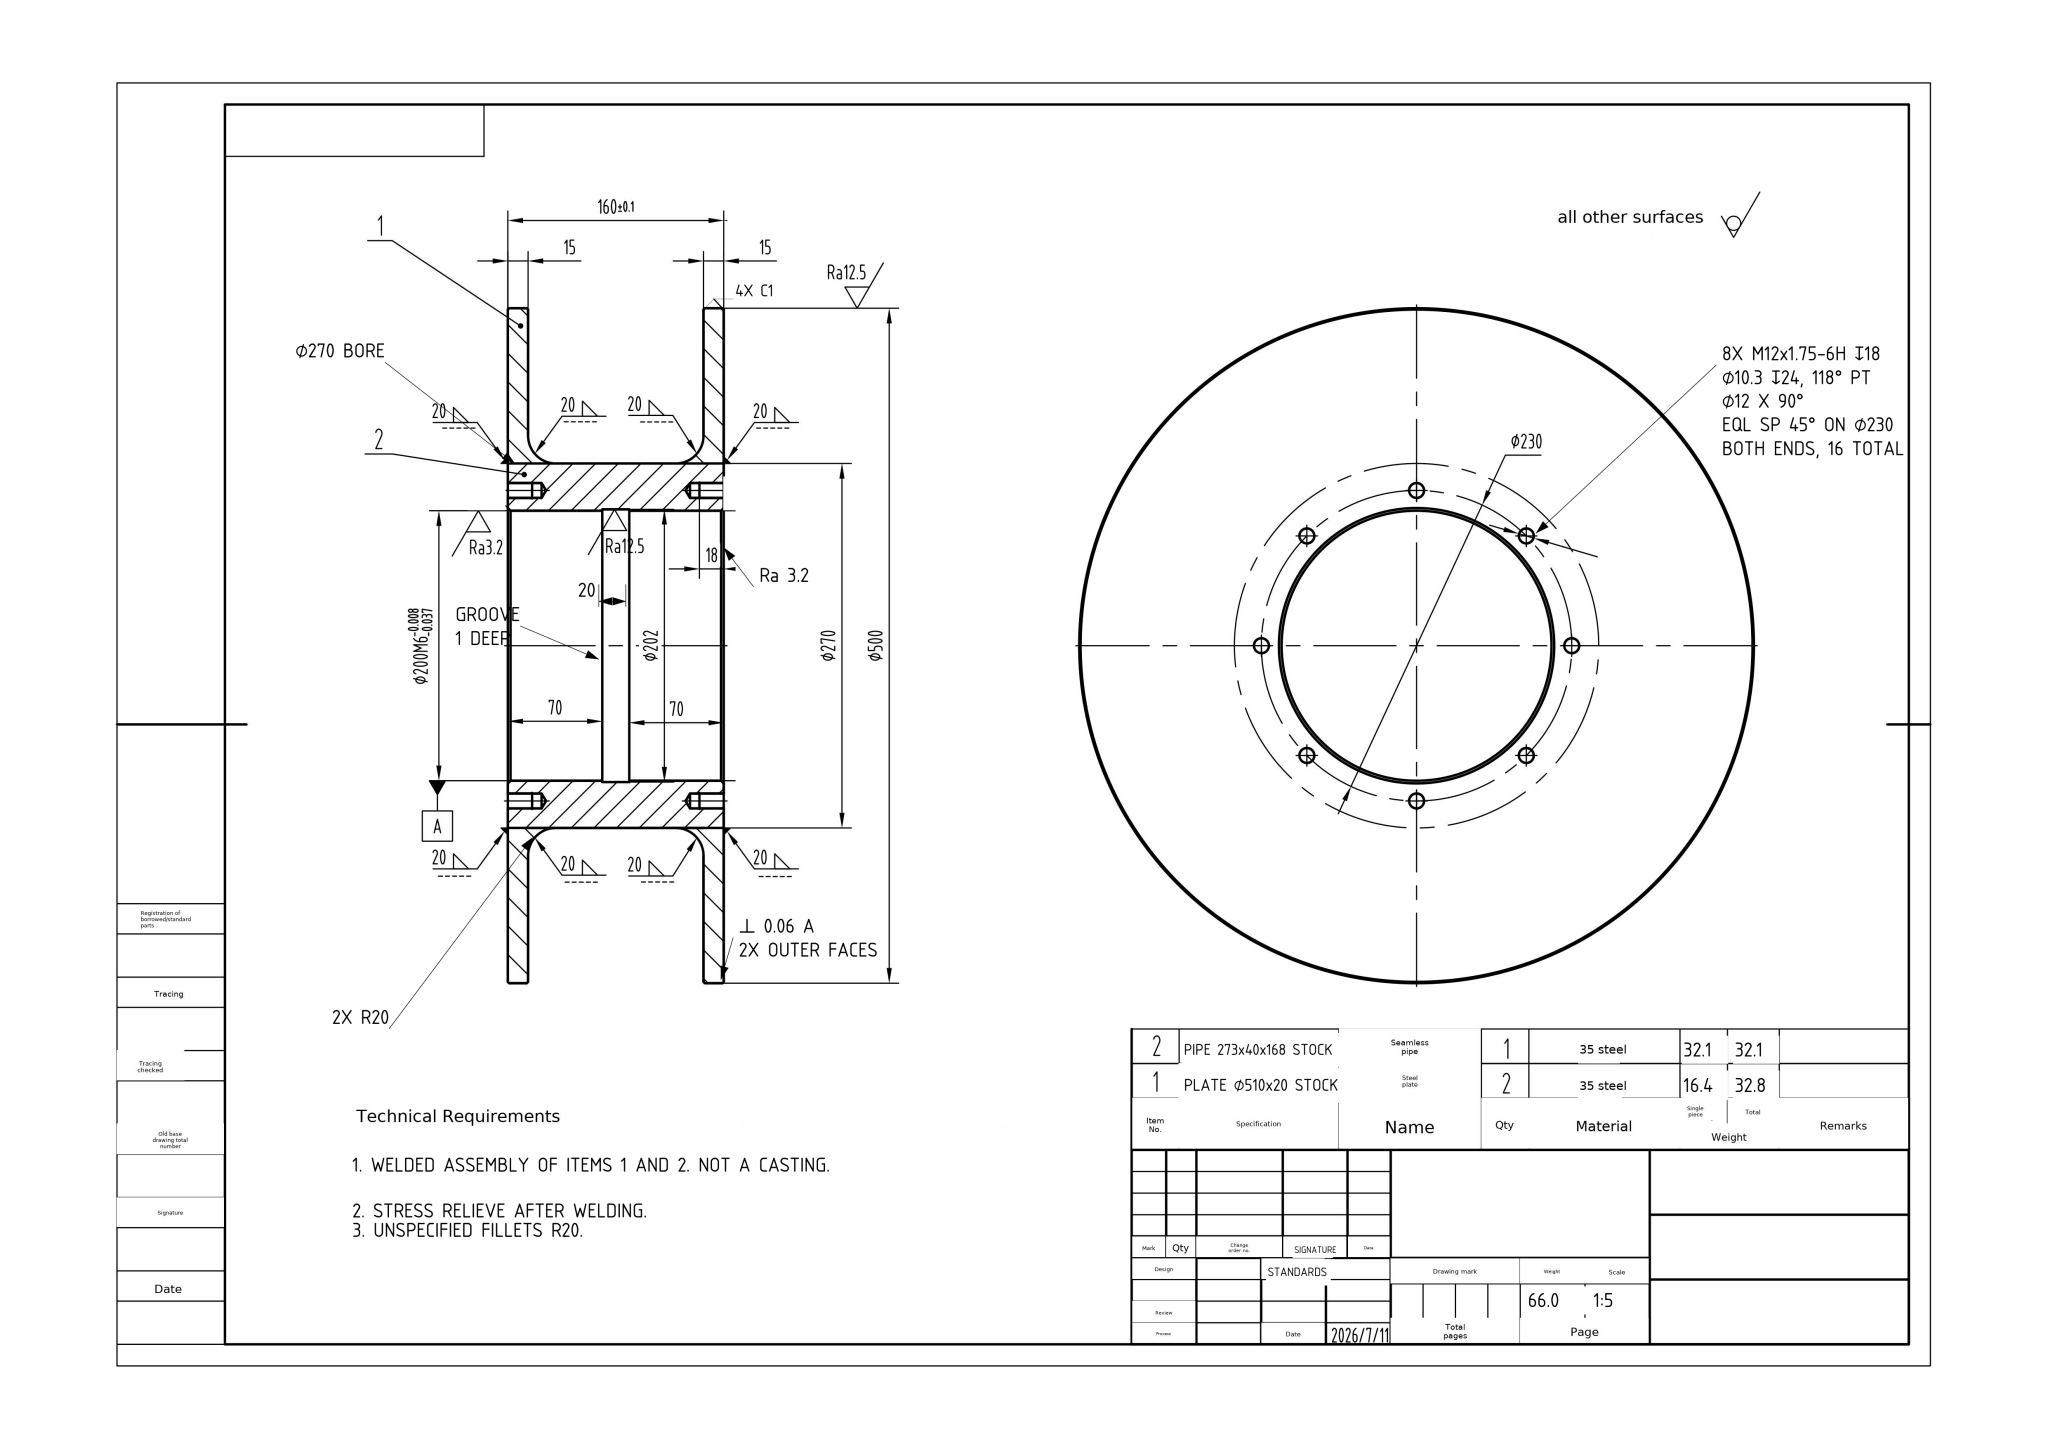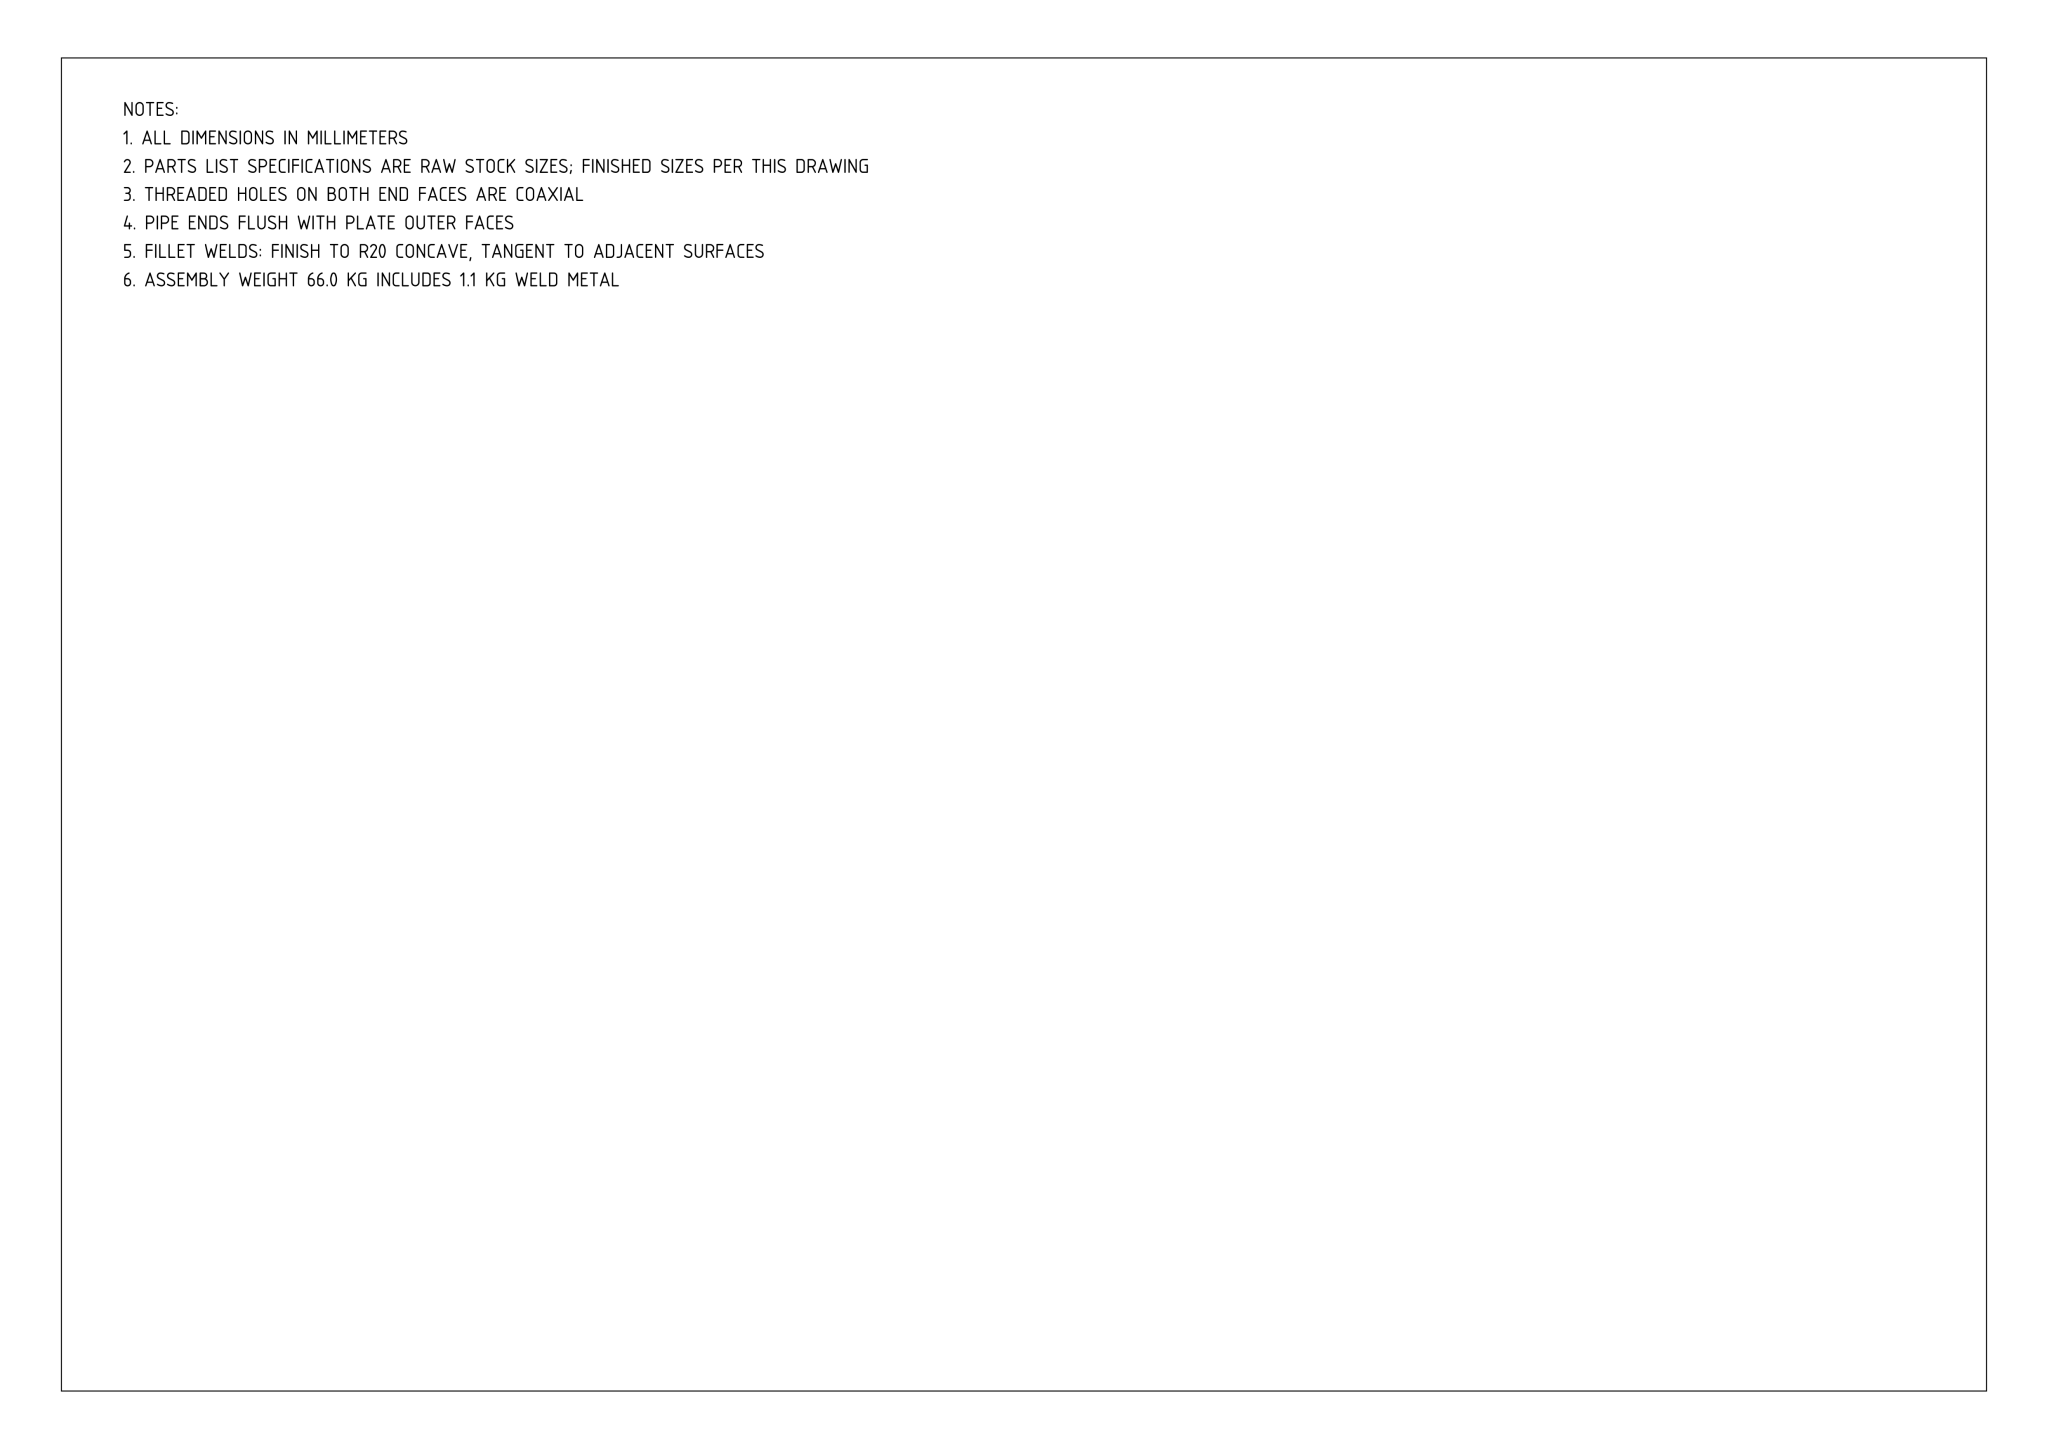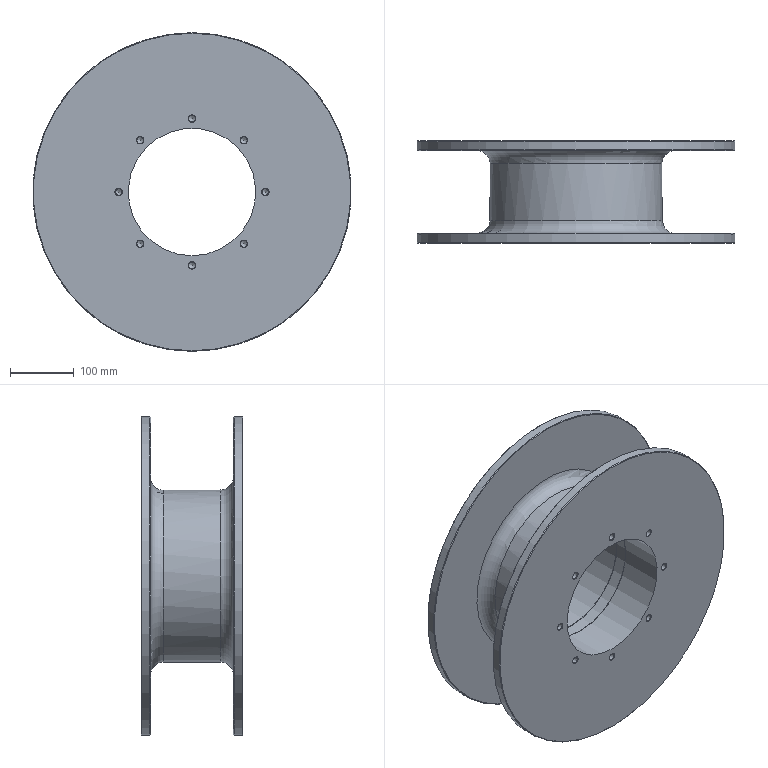Part | NX | mm | 1 solid | 66 faces | box 500 x 160 x 500 mm | volume 8408266 mm3 | cone 36 | cylinder 22 | plane 6 | torus 2 | commonest cylinder face diameters 10.3 x16 500 x2 200 x2 270 x1 202 x1